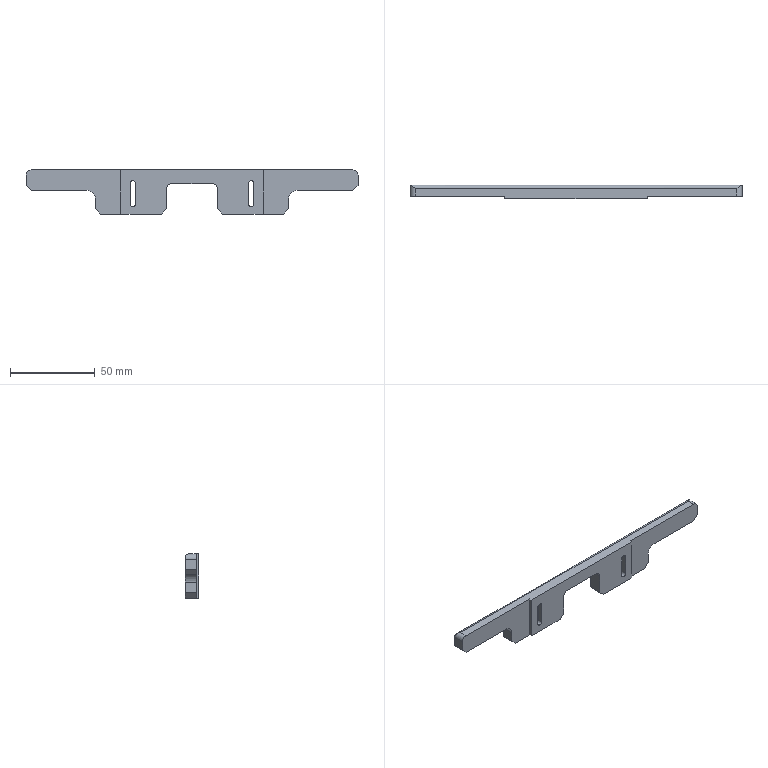Component | SolidWorks | SAWH02-03109A0RearPushBlock-3 | 1 solid | 49 faces | box 196 x 8 x 26 mm | volume 22836 mm3 | plane 34 | cylinder 15 | commonest cylinder face diameters 3.2 x4 7 x4 6 x4 10 x2 4 x1 | material Light Green Fiberglass Board